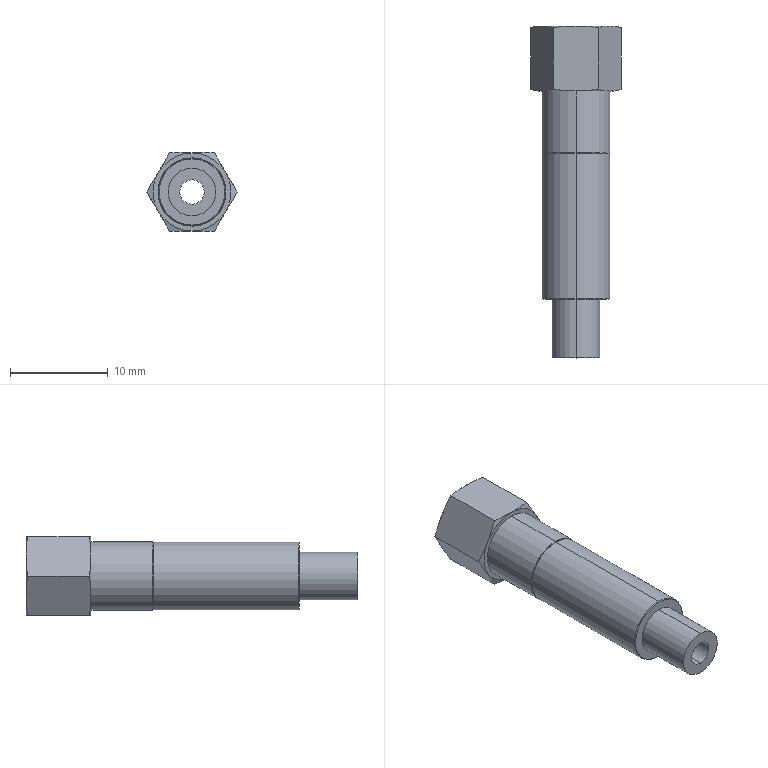Component | SolidWorks | ZPT06UNK6_B5_A80214-1_ZPT06U6_B5_B_BUFFER0214-1 | 1 solid | 41 faces | box 9.24 x 34 x 8 mm | volume 1077 mm3 | cone 20 | plane 11 | cylinder 10 | commonest cylinder face diameters 4.134 x2 7 x2 6.917 x2 4.9 x2 2.5 x2
build123d program:
from build123d import *

# Parameters (mm, degrees)
SKETCH2_R          = 8
CUT_EXTRUDE1_DEPTH = 6.65


with BuildPart() as part:
    # Sketch1 → Revolve1 (revolve)
    with BuildSketch(Plane.XY, mode=Mode.PRIVATE) as revolve1_sk:
        Polygon((1.25, 12), (2.45, 12), (2.45, 18), (3.386, 18), (3.458, 18.072), (3.458, 32.928), (3.386, 33), (3.5, 33), (3.5, 39.35), (4, 39.35), (6.4, 39.993), (6.4, 45.357), (4, 46), (2.5, 46), (2.067, 45.567), (2.067, 41), (1.25, 40.528), align=None)
    revolve(revolve1_sk.sketch.rotate(Axis((0, 12, 0), (0, 1, 0)), 270), axis=Axis((0, 12, 0), (0, 1, 0)))

    # Sketch2 → Cut-Extrude1 (cut)
    with BuildSketch(Plane(origin=(0, 46, 0), x_dir=(1, 0, 0), z_dir=(0, 1, 0))):
        Circle(SKETCH2_R)
        Polygon((-4.619, 0), (-2.309, -4), (2.309, -4), (4.619, 0), (2.309, 4), (-2.309, 4), align=None, mode=Mode.SUBTRACT)
    extrude(amount=-CUT_EXTRUDE1_DEPTH, mode=Mode.SUBTRACT)


solid = part.part

# Placed as in the assembly
solid = solid.moved(Location((-75, -83, 9.1), (0, 0, 0)))